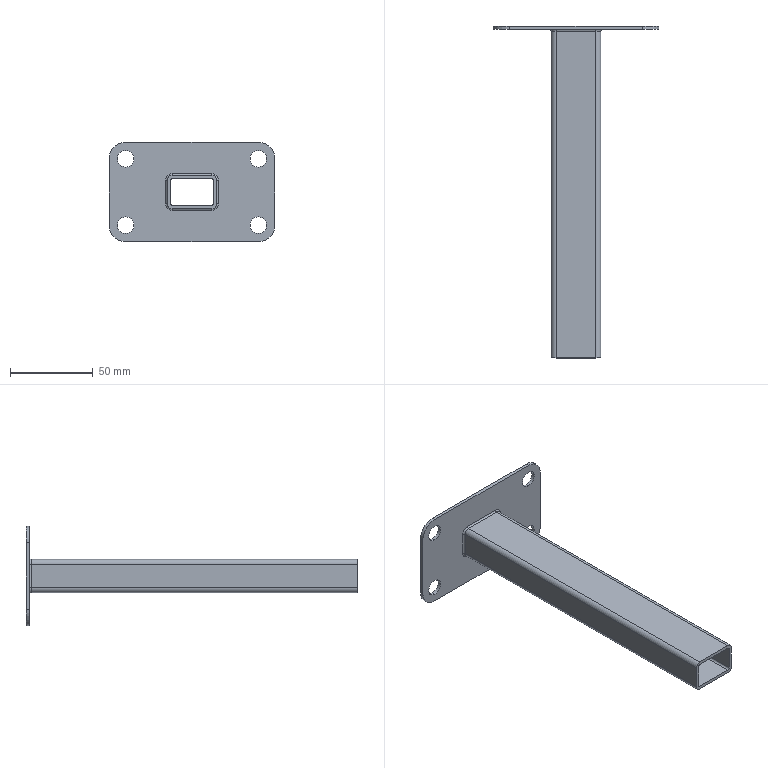Component | SolidWorks | CleaningRobotAssembly-1_A30x20x2RectangularColdFormedHollowSectionSteel300mm-1 | 1 solid | 51 faces | box 100 x 200 x 60 mm | volume 45445 mm3 | cylinder 28 | plane 15 | torus 8 | commonest cylinder face diameters 2 x12 10 x8 6 x4 20 x4
build123d program:
from build123d import *

# Parameters (mm, degrees)
BOSS_EXTRUDE1_DEPTH = 200
SKETCH2_W           = 60
SKETCH2_H           = 100
BOSS_EXTRUDE2_DEPTH = 2
FILLET1_R           = 1
FILLET2_R           = 1
FILLET3_R           = 10
SKETCH3_R           = 5
CUT_EXTRUDE1_DEPTH  = 28


with BuildPart() as part:
    # Sketch1 → Boss-Extrude1 (new body)
    with BuildSketch(Plane(origin=(0, 0, 0), x_dir=(0, 0, -1), z_dir=(1, 0, 0))):
        with BuildLine():
            Line((-6.263, 13), (6.263, 13))
            Line((6.263, 13), (7.561, 14.947))
            ThreePointArc((7.561, 14.947), (7.282, 14.987), (7, 15))
            Line((7, 15), (-7, 15))
            ThreePointArc((-7, 15), (-7.282, 14.987), (-7.561, 14.947))
            Line((-7.561, 14.947), (-6.263, 13))
        make_face()
        with BuildLine():
            Line((-10, -11.394), (-8, -8.394))
            Line((-8, -8.394), (-8, 12))
            ThreePointArc((-8, 12), (-7.707, 12.707), (-7, 13))
            Line((-7, 13), (-6.263, 13))
            Line((-6.263, 13), (-7.561, 14.947))
            ThreePointArc((-7.561, 14.947), (-9.311, 13.913), (-10, 12))
            Line((-10, 12), (-10, -11.394))
        make_face()
        with BuildLine():
            Line((8, 12), (8, -8.394))
            Line((8, -8.394), (10, -11.394))
            Line((10, -11.394), (10, 12))
            ThreePointArc((10, 12), (9.311, 13.913), (7.561, 14.947))
            Line((7.561, 14.947), (6.263, 13))
            Line((6.263, 13), (7, 13))
            ThreePointArc((7, 13), (7.707, 12.707), (8, 12))
        make_face()
        with BuildLine():
            Line((7, -13), (-7, -13))
            ThreePointArc((-7, -13), (-7.707, -12.707), (-8, -12))
            Line((-8, -12), (-8, -8.394))
            Line((-8, -8.394), (-10, -11.394))
            Line((-10, -11.394), (-10, -12))
            ThreePointArc((-10, -12), (-9.121, -14.121), (-7, -15))
            Line((-7, -15), (7, -15))
            ThreePointArc((7, -15), (9.121, -14.121), (10, -12))
            Line((10, -12), (10, -11.394))
            Line((10, -11.394), (8, -8.394))
            Line((8, -8.394), (8, -12))
            ThreePointArc((8, -12), (7.707, -12.707), (7, -13))
        make_face()
    extrude(amount=BOSS_EXTRUDE1_DEPTH)

    # Sketch2 → Boss-Extrude2 (add)
    with BuildSketch(Plane.ZY):
        Rectangle(SKETCH2_W, SKETCH2_H)
        with BuildLine():
            Line((-10, -12), (-10, 12))
            ThreePointArc((-10, 12), (-9.121, 14.121), (-7, 15))
            Line((-7, 15), (7, 15))
            ThreePointArc((7, 15), (9.121, 14.121), (10, 12))
            Line((10, 12), (10, -12))
            ThreePointArc((10, -12), (9.121, -14.121), (7, -15))
            Line((7, -15), (-7, -15))
            ThreePointArc((-7, -15), (-9.121, -14.121), (-10, -12))
        make_face(mode=Mode.SUBTRACT)
    extrude(amount=-BOSS_EXTRUDE2_DEPTH)

    # Fillet1
    fillet1_edges = [part.edges().sort_by_distance(p)[0] for p in [
        (2, 14.121, -9.121),
        (2, 0, -10),
        (2, -14.121, -9.121),
        (2, -15, 0),
        (2, -14.121, 9.121),
        (2, 0, 10),
        (2, 14.121, 9.121),
        (2, 15, 0),
    ]]
    fillet(fillet1_edges, radius=FILLET1_R)

    # Fillet2
    fillet2_edges = [part.edges().sort_by_distance(p)[0] for p in [
        (0, -13, 0),
        (0, -12.707, -7.707),
        (0, 0, -8),
        (0, 12.707, -7.707),
        (0, 13, 0),
        (0, 12.707, 7.707),
        (0, 0, 8),
        (0, -12.707, 7.707),
    ]]
    fillet(fillet2_edges, radius=FILLET2_R)

    # Fillet3
    fillet3_edges = [part.edges().sort_by_distance(p)[0] for p in [
        (1, 50, 30),
        (1, -50, 30),
        (1, -50, -30),
        (1, 50, -30),
    ]]
    fillet(fillet3_edges, radius=FILLET3_R)

    # Sketch3 → Cut-Extrude1 (cut)
    with BuildSketch(Plane.ZY):
        with Locations((-20, -40)):
            Circle(SKETCH3_R)
        with Locations((-20, 40)):
            Circle(SKETCH3_R)
        with Locations((20, 40)):
            Circle(SKETCH3_R)
        with Locations((20, -40)):
            Circle(SKETCH3_R)
    extrude(amount=-CUT_EXTRUDE1_DEPTH, mode=Mode.SUBTRACT)


solid = part.part

# Placed as in the assembly
solid = solid.moved(Location((310.629, -57.9, 228), (0, 0, -90)))